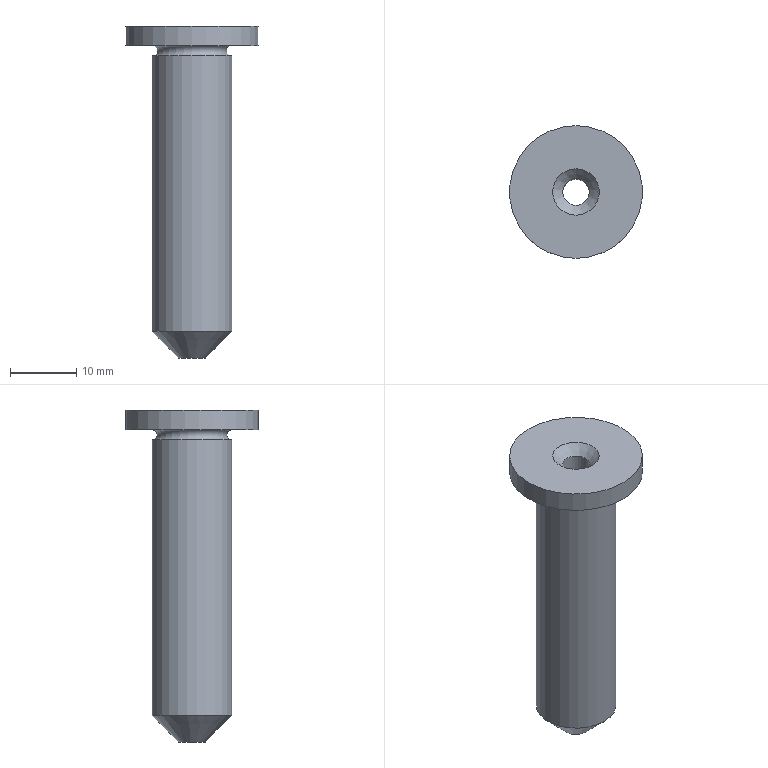Component | NX | COLLAR | 1 solid | 8 faces | box 20 x 20 x 50 mm | volume 5346 mm3 | cylinder 3 | cone 2 | plane 2 | torus 1 | commonest cylinder face diameters 4 x1 12 x1 20 x1
STEP:
#1=CARTESIAN_POINT('',(0.,0.,0.));
#2=DIRECTION('',(0.,0.,1.));
#3=DIRECTION('',(1.,0.,0.));
#4=AXIS2_PLACEMENT_3D('',#1,#2,#3);
#5=CARTESIAN_POINT('',(-146.777,2.,221.));
#6=VERTEX_POINT('',#5);
#7=CARTESIAN_POINT('',(-146.777,0.,221.));
#8=DIRECTION('',(0.,0.,-1.));
#9=DIRECTION('',(0.,1.,0.));
#10=AXIS2_PLACEMENT_3D('',#7,#8,#9);
#11=CIRCLE('',#10,2.);
#12=CARTESIAN_POINT('',(-146.777,0.,271.));
#13=DIRECTION('',(0.,0.,-1.));
#14=DIRECTION('',(0.,1.,0.));
#15=AXIS2_PLACEMENT_3D('',#12,#13,#14);
#16=CYLINDRICAL_SURFACE('',#15,2.);
#17=CARTESIAN_POINT('',(0.,50.));
#18=DIRECTION('',(1.,0.));
#19=VECTOR('',#18,1.);
#20=LINE('',#17,#19);
#21=(GEOMETRIC_REPRESENTATION_CONTEXT(2)PARAMETRIC_REPRESENTATION_CONTEXT()REPRESENTATION_CONTEXT('',''));
#22=DEFINITIONAL_REPRESENTATION('',(#20),#21);
#23=PCURVE('',#16,#22);
#24=CARTESIAN_POINT('',(-146.777,0.,221.));
#25=DIRECTION('',(0.,0.,1.));
#26=DIRECTION('',(0.,-1.,0.));
#27=AXIS2_PLACEMENT_3D('',#24,#25,#26);
#28=CONICAL_SURFACE('',#27,2.,0.7854);
#29=CARTESIAN_POINT('',(9.425,0.));
#30=DIRECTION('',(-1.,0.));
#31=VECTOR('',#30,1.);
#32=LINE('',#29,#31);
#33=(GEOMETRIC_REPRESENTATION_CONTEXT(2)PARAMETRIC_REPRESENTATION_CONTEXT()REPRESENTATION_CONTEXT('',''));
#34=DEFINITIONAL_REPRESENTATION('',(#32),#33);
#35=PCURVE('',#28,#34);
#36=SURFACE_CURVE('',#11,(#23,#35),.PCURVE_S1.);
#37=EDGE_CURVE('',#6,#6,#36,.T.);
#38=ORIENTED_EDGE('',*,*,#37,.F.);
#39=CARTESIAN_POINT('',(-146.777,2.,269.5));
#40=VERTEX_POINT('',#39);
#41=CARTESIAN_POINT('',(-146.777,2.,269.5));
#42=CARTESIAN_POINT('',(-146.777,2.,221.));
#43=B_SPLINE_CURVE_WITH_KNOTS('',1,(#41,#42),.UNSPECIFIED.,.F.,.F.,(2,2),(1.5,50.),.PIECEWISE_BEZIER_KNOTS.);
#44=CARTESIAN_POINT('',(0.,0.));
#45=DIRECTION('',(0.,1.));
#46=VECTOR('',#45,1.);
#47=LINE('',#44,#46);
#48=(GEOMETRIC_REPRESENTATION_CONTEXT(2)PARAMETRIC_REPRESENTATION_CONTEXT()REPRESENTATION_CONTEXT('',''));
#49=DEFINITIONAL_REPRESENTATION('',(#47),#48);
#50=PCURVE('',#16,#49);
#51=CARTESIAN_POINT('',(6.283,0.));
#52=DIRECTION('',(0.,1.));
#53=VECTOR('',#52,1.);
#54=LINE('',#51,#53);
#55=(GEOMETRIC_REPRESENTATION_CONTEXT(2)PARAMETRIC_REPRESENTATION_CONTEXT()REPRESENTATION_CONTEXT('',''));
#56=DEFINITIONAL_REPRESENTATION('',(#54),#55);
#57=PCURVE('',#16,#56);
#58=SEAM_CURVE('',#43,(#50,#57),.PCURVE_S1.);
#59=EDGE_CURVE('',#40,#6,#58,.T.);
#60=ORIENTED_EDGE('',*,*,#59,.F.);
#61=CARTESIAN_POINT('',(-146.777,0.,269.5));
#62=DIRECTION('',(0.,0.,-1.));
#63=DIRECTION('',(0.,1.,0.));
#64=AXIS2_PLACEMENT_3D('',#61,#62,#63);
#65=CIRCLE('',#64,2.);
#66=CARTESIAN_POINT('',(0.,1.5));
#67=DIRECTION('',(1.,0.));
#68=VECTOR('',#67,1.);
#69=LINE('',#66,#68);
#70=(GEOMETRIC_REPRESENTATION_CONTEXT(2)PARAMETRIC_REPRESENTATION_CONTEXT()REPRESENTATION_CONTEXT('',''));
#71=DEFINITIONAL_REPRESENTATION('',(#69),#70);
#72=PCURVE('',#16,#71);
#73=CARTESIAN_POINT('',(-146.777,0.,271.));
#74=DIRECTION('',(0.,0.,1.));
#75=DIRECTION('',(0.,-1.,0.));
#76=AXIS2_PLACEMENT_3D('',#73,#74,#75);
#77=CONICAL_SURFACE('',#76,3.5,0.7854);
#78=CARTESIAN_POINT('',(9.425,-1.5));
#79=DIRECTION('',(-1.,0.));
#80=VECTOR('',#79,1.);
#81=LINE('',#78,#80);
#82=(GEOMETRIC_REPRESENTATION_CONTEXT(2)PARAMETRIC_REPRESENTATION_CONTEXT()REPRESENTATION_CONTEXT('',''));
#83=DEFINITIONAL_REPRESENTATION('',(#81),#82);
#84=PCURVE('',#77,#83);
#85=SURFACE_CURVE('',#65,(#72,#84),.PCURVE_S1.);
#86=EDGE_CURVE('',#40,#40,#85,.T.);
#87=ORIENTED_EDGE('',*,*,#86,.T.);
#88=ORIENTED_EDGE('',*,*,#59,.T.);
#89=EDGE_LOOP('',(#38,#60,#87,#88));
#90=FACE_BOUND('',#89,.F.);
#91=ADVANCED_FACE('',(#90),#16,.F.);
#92=CARTESIAN_POINT('',(-146.777,6.,225.));
#93=VERTEX_POINT('',#92);
#94=CARTESIAN_POINT('',(-146.777,0.,225.));
#95=DIRECTION('',(0.,0.,-1.));
#96=DIRECTION('',(0.,1.,0.));
#97=AXIS2_PLACEMENT_3D('',#94,#95,#96);
#98=CIRCLE('',#97,6.);
#99=CARTESIAN_POINT('',(9.425,4.));
#100=DIRECTION('',(-1.,0.));
#101=VECTOR('',#100,1.);
#102=LINE('',#99,#101);
#103=(GEOMETRIC_REPRESENTATION_CONTEXT(2)PARAMETRIC_REPRESENTATION_CONTEXT()REPRESENTATION_CONTEXT('',''));
#104=DEFINITIONAL_REPRESENTATION('',(#102),#103);
#105=PCURVE('',#28,#104);
#106=CARTESIAN_POINT('',(-146.777,0.,271.));
#107=DIRECTION('',(0.,0.,-1.));
#108=DIRECTION('',(0.,1.,0.));
#109=AXIS2_PLACEMENT_3D('',#106,#107,#108);
#110=CYLINDRICAL_SURFACE('',#109,6.);
#111=CARTESIAN_POINT('',(0.,46.));
#112=DIRECTION('',(1.,0.));
#113=VECTOR('',#112,1.);
#114=LINE('',#111,#113);
#115=(GEOMETRIC_REPRESENTATION_CONTEXT(2)PARAMETRIC_REPRESENTATION_CONTEXT()REPRESENTATION_CONTEXT('',''));
#116=DEFINITIONAL_REPRESENTATION('',(#114),#115);
#117=PCURVE('',#110,#116);
#118=SURFACE_CURVE('',#98,(#105,#117),.PCURVE_S1.);
#119=EDGE_CURVE('',#93,#93,#118,.T.);
#120=ORIENTED_EDGE('',*,*,#119,.T.);
#121=CARTESIAN_POINT('',(-146.777,2.,221.));
#122=CARTESIAN_POINT('',(-146.777,6.,225.));
#123=B_SPLINE_CURVE_WITH_KNOTS('',1,(#121,#122),.UNSPECIFIED.,.F.,.F.,(2,2),(0.,5.657),.PIECEWISE_BEZIER_KNOTS.);
#124=CARTESIAN_POINT('',(3.142,0.));
#125=DIRECTION('',(0.,1.));
#126=VECTOR('',#125,1.);
#127=LINE('',#124,#126);
#128=(GEOMETRIC_REPRESENTATION_CONTEXT(2)PARAMETRIC_REPRESENTATION_CONTEXT()REPRESENTATION_CONTEXT('',''));
#129=DEFINITIONAL_REPRESENTATION('',(#127),#128);
#130=PCURVE('',#28,#129);
#131=CARTESIAN_POINT('',(9.425,0.));
#132=DIRECTION('',(0.,1.));
#133=VECTOR('',#132,1.);
#134=LINE('',#131,#133);
#135=(GEOMETRIC_REPRESENTATION_CONTEXT(2)PARAMETRIC_REPRESENTATION_CONTEXT()REPRESENTATION_CONTEXT('',''));
#136=DEFINITIONAL_REPRESENTATION('',(#134),#135);
#137=PCURVE('',#28,#136);
#138=SEAM_CURVE('',#123,(#130,#137),.PCURVE_S1.);
#139=EDGE_CURVE('',#6,#93,#138,.T.);
#140=ORIENTED_EDGE('',*,*,#139,.F.);
#141=ORIENTED_EDGE('',*,*,#37,.F.);
#142=ORIENTED_EDGE('',*,*,#139,.T.);
#143=EDGE_LOOP('',(#120,#140,#141,#142));
#144=FACE_BOUND('',#143,.T.);
#145=ADVANCED_FACE('',(#144),#28,.T.);
#146=CARTESIAN_POINT('',(-146.777,6.,266.5));
#147=VERTEX_POINT('',#146);
#148=CARTESIAN_POINT('',(-146.777,0.,266.5));
#149=DIRECTION('',(0.,0.,-1.));
#150=DIRECTION('',(0.,1.,0.));
#151=AXIS2_PLACEMENT_3D('',#148,#149,#150);
#152=CIRCLE('',#151,6.);
#153=CARTESIAN_POINT('',(0.,4.5));
#154=DIRECTION('',(1.,0.));
#155=VECTOR('',#154,1.);
#156=LINE('',#153,#155);
#157=(GEOMETRIC_REPRESENTATION_CONTEXT(2)PARAMETRIC_REPRESENTATION_CONTEXT()REPRESENTATION_CONTEXT('',''));
#158=DEFINITIONAL_REPRESENTATION('',(#156),#157);
#159=PCURVE('',#110,#158);
#160=CARTESIAN_POINT('',(-146.777,0.,267.25));
#161=DIRECTION('',(0.,0.,-1.));
#162=DIRECTION('',(0.,1.,0.));
#163=AXIS2_PLACEMENT_3D('',#160,#161,#162);
#164=TOROIDAL_SURFACE('',#163,6.,0.75);
#165=CARTESIAN_POINT('',(0.,1.571));
#166=DIRECTION('',(1.,0.));
#167=VECTOR('',#166,1.);
#168=LINE('',#165,#167);
#169=(GEOMETRIC_REPRESENTATION_CONTEXT(2)PARAMETRIC_REPRESENTATION_CONTEXT()REPRESENTATION_CONTEXT('',''));
#170=DEFINITIONAL_REPRESENTATION('',(#168),#169);
#171=PCURVE('',#164,#170);
#172=SURFACE_CURVE('',#152,(#159,#171),.PCURVE_S1.);
#173=EDGE_CURVE('',#147,#147,#172,.T.);
#174=ORIENTED_EDGE('',*,*,#173,.T.);
#175=CARTESIAN_POINT('',(-146.777,6.,266.5));
#176=CARTESIAN_POINT('',(-146.777,6.,225.));
#177=B_SPLINE_CURVE_WITH_KNOTS('',1,(#175,#176),.UNSPECIFIED.,.F.,.F.,(2,2),(4.5,46.),.PIECEWISE_BEZIER_KNOTS.);
#178=CARTESIAN_POINT('',(6.283,0.));
#179=DIRECTION('',(0.,1.));
#180=VECTOR('',#179,1.);
#181=LINE('',#178,#180);
#182=(GEOMETRIC_REPRESENTATION_CONTEXT(2)PARAMETRIC_REPRESENTATION_CONTEXT()REPRESENTATION_CONTEXT('',''));
#183=DEFINITIONAL_REPRESENTATION('',(#181),#182);
#184=PCURVE('',#110,#183);
#185=CARTESIAN_POINT('',(0.,0.));
#186=DIRECTION('',(0.,1.));
#187=VECTOR('',#186,1.);
#188=LINE('',#185,#187);
#189=(GEOMETRIC_REPRESENTATION_CONTEXT(2)PARAMETRIC_REPRESENTATION_CONTEXT()REPRESENTATION_CONTEXT('',''));
#190=DEFINITIONAL_REPRESENTATION('',(#188),#189);
#191=PCURVE('',#110,#190);
#192=SEAM_CURVE('',#177,(#184,#191),.PCURVE_S1.);
#193=EDGE_CURVE('',#147,#93,#192,.T.);
#194=ORIENTED_EDGE('',*,*,#193,.T.);
#195=ORIENTED_EDGE('',*,*,#119,.F.);
#196=ORIENTED_EDGE('',*,*,#193,.F.);
#197=EDGE_LOOP('',(#174,#194,#195,#196));
#198=FACE_BOUND('',#197,.T.);
#199=ADVANCED_FACE('',(#198),#110,.T.);
#200=CARTESIAN_POINT('',(-146.777,6.,268.));
#201=VERTEX_POINT('',#200);
#202=CARTESIAN_POINT('',(-146.777,0.,268.));
#203=DIRECTION('',(0.,0.,-1.));
#204=DIRECTION('',(0.,1.,0.));
#205=AXIS2_PLACEMENT_3D('',#202,#203,#204);
#206=CIRCLE('',#205,6.);
#207=CARTESIAN_POINT('',(0.,4.712));
#208=DIRECTION('',(1.,0.));
#209=VECTOR('',#208,1.);
#210=LINE('',#207,#209);
#211=(GEOMETRIC_REPRESENTATION_CONTEXT(2)PARAMETRIC_REPRESENTATION_CONTEXT()REPRESENTATION_CONTEXT('',''));
#212=DEFINITIONAL_REPRESENTATION('',(#210),#211);
#213=PCURVE('',#164,#212);
#214=CARTESIAN_POINT('',(-140.777,0.,268.));
#215=DIRECTION('',(0.,0.,-1.));
#216=DIRECTION('',(0.,1.,0.));
#217=AXIS2_PLACEMENT_3D('',#214,#215,#216);
#218=PLANE('',#217);
#219=CARTESIAN_POINT('',(0.,-6.));
#220=DIRECTION('',(1.,0.));
#221=AXIS2_PLACEMENT_2D('',#219,#220);
#222=CIRCLE('',#221,6.);
#223=(GEOMETRIC_REPRESENTATION_CONTEXT(2)PARAMETRIC_REPRESENTATION_CONTEXT()REPRESENTATION_CONTEXT('',''));
#224=DEFINITIONAL_REPRESENTATION('',(#222),#223);
#225=PCURVE('',#218,#224);
#226=SURFACE_CURVE('',#206,(#213,#225),.PCURVE_S1.);
#227=EDGE_CURVE('',#201,#201,#226,.T.);
#228=ORIENTED_EDGE('',*,*,#227,.F.);
#229=CARTESIAN_POINT('',(-146.777,6.,266.5));
#230=CARTESIAN_POINT('',(-146.777,5.705,266.5));
#231=CARTESIAN_POINT('',(-146.777,5.411,266.632));
#232=CARTESIAN_POINT('',(-146.777,5.186,266.896));
#233=CARTESIAN_POINT('',(-146.777,5.099,267.25));
#234=CARTESIAN_POINT('',(-146.777,5.186,267.604));
#235=CARTESIAN_POINT('',(-146.777,5.411,267.868));
#236=CARTESIAN_POINT('',(-146.777,5.705,268.));
#237=CARTESIAN_POINT('',(-146.777,6.,268.));
#238=B_SPLINE_CURVE_WITH_KNOTS('',8,(#229,#230,#231,#232,#233,#234,#235,#236,#237),.UNSPECIFIED.,.F.,.F.,(9,9),(1.571,4.712),.PIECEWISE_BEZIER_KNOTS.);
#239=CARTESIAN_POINT('',(0.,0.));
#240=DIRECTION('',(0.,1.));
#241=VECTOR('',#240,1.);
#242=LINE('',#239,#241);
#243=(GEOMETRIC_REPRESENTATION_CONTEXT(2)PARAMETRIC_REPRESENTATION_CONTEXT()REPRESENTATION_CONTEXT('',''));
#244=DEFINITIONAL_REPRESENTATION('',(#242),#243);
#245=PCURVE('',#164,#244);
#246=CARTESIAN_POINT('',(6.283,0.));
#247=DIRECTION('',(0.,1.));
#248=VECTOR('',#247,1.);
#249=LINE('',#246,#248);
#250=(GEOMETRIC_REPRESENTATION_CONTEXT(2)PARAMETRIC_REPRESENTATION_CONTEXT()REPRESENTATION_CONTEXT('',''));
#251=DEFINITIONAL_REPRESENTATION('',(#249),#250);
#252=PCURVE('',#164,#251);
#253=SEAM_CURVE('',#238,(#245,#252),.PCURVE_S1.);
#254=EDGE_CURVE('',#147,#201,#253,.T.);
#255=ORIENTED_EDGE('',*,*,#254,.F.);
#256=ORIENTED_EDGE('',*,*,#173,.T.);
#257=ORIENTED_EDGE('',*,*,#254,.T.);
#258=EDGE_LOOP('',(#228,#255,#256,#257));
#259=FACE_BOUND('',#258,.F.);
#260=ADVANCED_FACE('',(#259),#164,.F.);
#261=CARTESIAN_POINT('',(-146.777,10.,268.));
#262=VERTEX_POINT('',#261);
#263=CARTESIAN_POINT('',(-146.777,0.,268.));
#264=DIRECTION('',(0.,0.,-1.));
#265=DIRECTION('',(0.,1.,0.));
#266=AXIS2_PLACEMENT_3D('',#263,#264,#265);
#267=CIRCLE('',#266,10.);
#268=CARTESIAN_POINT('',(0.,-6.));
#269=DIRECTION('',(1.,0.));
#270=AXIS2_PLACEMENT_2D('',#268,#269);
#271=CIRCLE('',#270,10.);
#272=(GEOMETRIC_REPRESENTATION_CONTEXT(2)PARAMETRIC_REPRESENTATION_CONTEXT()REPRESENTATION_CONTEXT('',''));
#273=DEFINITIONAL_REPRESENTATION('',(#271),#272);
#274=PCURVE('',#218,#273);
#275=CARTESIAN_POINT('',(-146.777,0.,271.));
#276=DIRECTION('',(0.,0.,-1.));
#277=DIRECTION('',(0.,1.,0.));
#278=AXIS2_PLACEMENT_3D('',#275,#276,#277);
#279=CYLINDRICAL_SURFACE('',#278,10.);
#280=CARTESIAN_POINT('',(0.,3.));
#281=DIRECTION('',(1.,0.));
#282=VECTOR('',#281,1.);
#283=LINE('',#280,#282);
#284=(GEOMETRIC_REPRESENTATION_CONTEXT(2)PARAMETRIC_REPRESENTATION_CONTEXT()REPRESENTATION_CONTEXT('',''));
#285=DEFINITIONAL_REPRESENTATION('',(#283),#284);
#286=PCURVE('',#279,#285);
#287=SURFACE_CURVE('',#267,(#274,#286),.PCURVE_S1.);
#288=EDGE_CURVE('',#262,#262,#287,.T.);
#289=ORIENTED_EDGE('',*,*,#288,.T.);
#290=EDGE_LOOP('',(#289));
#291=FACE_BOUND('',#290,.T.);
#292=ORIENTED_EDGE('',*,*,#227,.F.);
#293=EDGE_LOOP('',(#292));
#294=FACE_BOUND('',#293,.T.);
#295=ADVANCED_FACE('',(#291,#294),#218,.T.);
#296=CARTESIAN_POINT('',(-146.777,10.,271.));
#297=VERTEX_POINT('',#296);
#298=CARTESIAN_POINT('',(-146.777,0.,271.));
#299=DIRECTION('',(0.,0.,-1.));
#300=DIRECTION('',(0.,1.,0.));
#301=AXIS2_PLACEMENT_3D('',#298,#299,#300);
#302=CIRCLE('',#301,10.);
#303=CARTESIAN_POINT('',(0.,0.));
#304=DIRECTION('',(1.,0.));
#305=VECTOR('',#304,1.);
#306=LINE('',#303,#305);
#307=(GEOMETRIC_REPRESENTATION_CONTEXT(2)PARAMETRIC_REPRESENTATION_CONTEXT()REPRESENTATION_CONTEXT('',''));
#308=DEFINITIONAL_REPRESENTATION('',(#306),#307);
#309=PCURVE('',#279,#308);
#310=CARTESIAN_POINT('',(-136.777,0.,271.));
#311=DIRECTION('',(0.,0.,1.));
#312=DIRECTION('',(0.,-1.,0.));
#313=AXIS2_PLACEMENT_3D('',#310,#311,#312);
#314=PLANE('',#313);
#315=CARTESIAN_POINT('',(-10.,-10.));
#316=CARTESIAN_POINT('',(-10.,7.321));
#317=CARTESIAN_POINT('',(5.,-1.34));
#318=CARTESIAN_POINT('',(20.,-10.));
#319=CARTESIAN_POINT('',(5.,-18.66));
#320=CARTESIAN_POINT('',(-10.,-27.321));
#321=CARTESIAN_POINT('',(-10.,-10.));
#322=(BOUNDED_CURVE()B_SPLINE_CURVE(2,(#315,#316,#317,#318,#319,#320,#321),.UNSPECIFIED.,.T.,.F.)B_SPLINE_CURVE_WITH_KNOTS((1,2,2,2,2,1),(-2.094,0.,2.094,4.189,6.283,8.378),.UNSPECIFIED.)CURVE()GEOMETRIC_REPRESENTATION_ITEM()RATIONAL_B_SPLINE_CURVE((1.,0.5,1.,0.5,1.,0.5,1.))REPRESENTATION_ITEM(''));
#323=(GEOMETRIC_REPRESENTATION_CONTEXT(2)PARAMETRIC_REPRESENTATION_CONTEXT()REPRESENTATION_CONTEXT('',''));
#324=DEFINITIONAL_REPRESENTATION('',(#322),#323);
#325=PCURVE('',#314,#324);
#326=SURFACE_CURVE('',#302,(#309,#325),.PCURVE_S1.);
#327=EDGE_CURVE('',#297,#297,#326,.T.);
#328=ORIENTED_EDGE('',*,*,#327,.T.);
#329=CARTESIAN_POINT('',(-146.777,10.,271.));
#330=CARTESIAN_POINT('',(-146.777,10.,268.));
#331=B_SPLINE_CURVE_WITH_KNOTS('',1,(#329,#330),.UNSPECIFIED.,.F.,.F.,(2,2),(0.,3.),.PIECEWISE_BEZIER_KNOTS.);
#332=CARTESIAN_POINT('',(6.283,0.));
#333=DIRECTION('',(0.,1.));
#334=VECTOR('',#333,1.);
#335=LINE('',#332,#334);
#336=(GEOMETRIC_REPRESENTATION_CONTEXT(2)PARAMETRIC_REPRESENTATION_CONTEXT()REPRESENTATION_CONTEXT('',''));
#337=DEFINITIONAL_REPRESENTATION('',(#335),#336);
#338=PCURVE('',#279,#337);
#339=CARTESIAN_POINT('',(0.,0.));
#340=DIRECTION('',(0.,1.));
#341=VECTOR('',#340,1.);
#342=LINE('',#339,#341);
#343=(GEOMETRIC_REPRESENTATION_CONTEXT(2)PARAMETRIC_REPRESENTATION_CONTEXT()REPRESENTATION_CONTEXT('',''));
#344=DEFINITIONAL_REPRESENTATION('',(#342),#343);
#345=PCURVE('',#279,#344);
#346=SEAM_CURVE('',#331,(#338,#345),.PCURVE_S1.);
#347=EDGE_CURVE('',#297,#262,#346,.T.);
#348=ORIENTED_EDGE('',*,*,#347,.T.);
#349=ORIENTED_EDGE('',*,*,#288,.F.);
#350=ORIENTED_EDGE('',*,*,#347,.F.);
#351=EDGE_LOOP('',(#328,#348,#349,#350));
#352=FACE_BOUND('',#351,.T.);
#353=ADVANCED_FACE('',(#352),#279,.T.);
#354=CARTESIAN_POINT('',(-146.777,3.5,271.));
#355=VERTEX_POINT('',#354);
#356=CARTESIAN_POINT('',(-146.777,0.,271.));
#357=DIRECTION('',(0.,0.,-1.));
#358=DIRECTION('',(0.,1.,0.));
#359=AXIS2_PLACEMENT_3D('',#356,#357,#358);
#360=CIRCLE('',#359,3.5);
#361=CARTESIAN_POINT('',(-3.5,-10.));
#362=CARTESIAN_POINT('',(-3.5,-3.938));
#363=CARTESIAN_POINT('',(1.75,-6.969));
#364=CARTESIAN_POINT('',(7.,-10.));
#365=CARTESIAN_POINT('',(1.75,-13.031));
#366=CARTESIAN_POINT('',(-3.5,-16.062));
#367=CARTESIAN_POINT('',(-3.5,-10.));
#368=(BOUNDED_CURVE()B_SPLINE_CURVE(2,(#361,#362,#363,#364,#365,#366,#367),.UNSPECIFIED.,.T.,.F.)B_SPLINE_CURVE_WITH_KNOTS((1,2,2,2,2,1),(-2.094,0.,2.094,4.189,6.283,8.378),.UNSPECIFIED.)CURVE()GEOMETRIC_REPRESENTATION_ITEM()RATIONAL_B_SPLINE_CURVE((1.,0.5,1.,0.5,1.,0.5,1.))REPRESENTATION_ITEM(''));
#369=(GEOMETRIC_REPRESENTATION_CONTEXT(2)PARAMETRIC_REPRESENTATION_CONTEXT()REPRESENTATION_CONTEXT('',''));
#370=DEFINITIONAL_REPRESENTATION('',(#368),#369);
#371=PCURVE('',#314,#370);
#372=CARTESIAN_POINT('',(9.425,0.));
#373=DIRECTION('',(-1.,0.));
#374=VECTOR('',#373,1.);
#375=LINE('',#372,#374);
#376=(GEOMETRIC_REPRESENTATION_CONTEXT(2)PARAMETRIC_REPRESENTATION_CONTEXT()REPRESENTATION_CONTEXT('',''));
#377=DEFINITIONAL_REPRESENTATION('',(#375),#376);
#378=PCURVE('',#77,#377);
#379=SURFACE_CURVE('',#360,(#371,#378),.PCURVE_S1.);
#380=EDGE_CURVE('',#355,#355,#379,.T.);
#381=ORIENTED_EDGE('',*,*,#380,.T.);
#382=EDGE_LOOP('',(#381));
#383=FACE_BOUND('',#382,.T.);
#384=ORIENTED_EDGE('',*,*,#327,.F.);
#385=EDGE_LOOP('',(#384));
#386=FACE_BOUND('',#385,.T.);
#387=ADVANCED_FACE('',(#383,#386),#314,.T.);
#388=ORIENTED_EDGE('',*,*,#86,.F.);
#389=CARTESIAN_POINT('',(-146.777,2.,269.5));
#390=CARTESIAN_POINT('',(-146.777,3.5,271.));
#391=B_SPLINE_CURVE_WITH_KNOTS('',1,(#389,#390),.UNSPECIFIED.,.F.,.F.,(2,2),(-2.121,0.),.PIECEWISE_BEZIER_KNOTS.);
#392=CARTESIAN_POINT('',(9.425,0.));
#393=DIRECTION('',(0.,1.));
#394=VECTOR('',#393,1.);
#395=LINE('',#392,#394);
#396=(GEOMETRIC_REPRESENTATION_CONTEXT(2)PARAMETRIC_REPRESENTATION_CONTEXT()REPRESENTATION_CONTEXT('',''));
#397=DEFINITIONAL_REPRESENTATION('',(#395),#396);
#398=PCURVE('',#77,#397);
#399=CARTESIAN_POINT('',(3.142,0.));
#400=DIRECTION('',(0.,1.));
#401=VECTOR('',#400,1.);
#402=LINE('',#399,#401);
#403=(GEOMETRIC_REPRESENTATION_CONTEXT(2)PARAMETRIC_REPRESENTATION_CONTEXT()REPRESENTATION_CONTEXT('',''));
#404=DEFINITIONAL_REPRESENTATION('',(#402),#403);
#405=PCURVE('',#77,#404);
#406=SEAM_CURVE('',#391,(#398,#405),.PCURVE_S1.);
#407=EDGE_CURVE('',#40,#355,#406,.T.);
#408=ORIENTED_EDGE('',*,*,#407,.T.);
#409=ORIENTED_EDGE('',*,*,#380,.T.);
#410=ORIENTED_EDGE('',*,*,#407,.F.);
#411=EDGE_LOOP('',(#388,#408,#409,#410));
#412=FACE_BOUND('',#411,.F.);
#413=ADVANCED_FACE('',(#412),#77,.F.);
#414=CLOSED_SHELL('',(#91,#145,#199,#260,#295,#353,#387,#413));
#415=MANIFOLD_SOLID_BREP('',#414);
#416=(LENGTH_UNIT()NAMED_UNIT(*)SI_UNIT(.MILLI.,.METRE.));
#417=UNCERTAINTY_MEASURE_WITH_UNIT(LENGTH_MEASURE(0.00001),#416,'','');
#418=(NAMED_UNIT(*)PLANE_ANGLE_UNIT()SI_UNIT($,.RADIAN.));
#419=(NAMED_UNIT(*)SI_UNIT($,.STERADIAN.)SOLID_ANGLE_UNIT());
#420=(GEOMETRIC_REPRESENTATION_CONTEXT(3)GLOBAL_UNCERTAINTY_ASSIGNED_CONTEXT((#417))GLOBAL_UNIT_ASSIGNED_CONTEXT((#416,#418,#419))REPRESENTATION_CONTEXT('',''));
#421=ADVANCED_BREP_SHAPE_REPRESENTATION('',(#4,#415),#420);